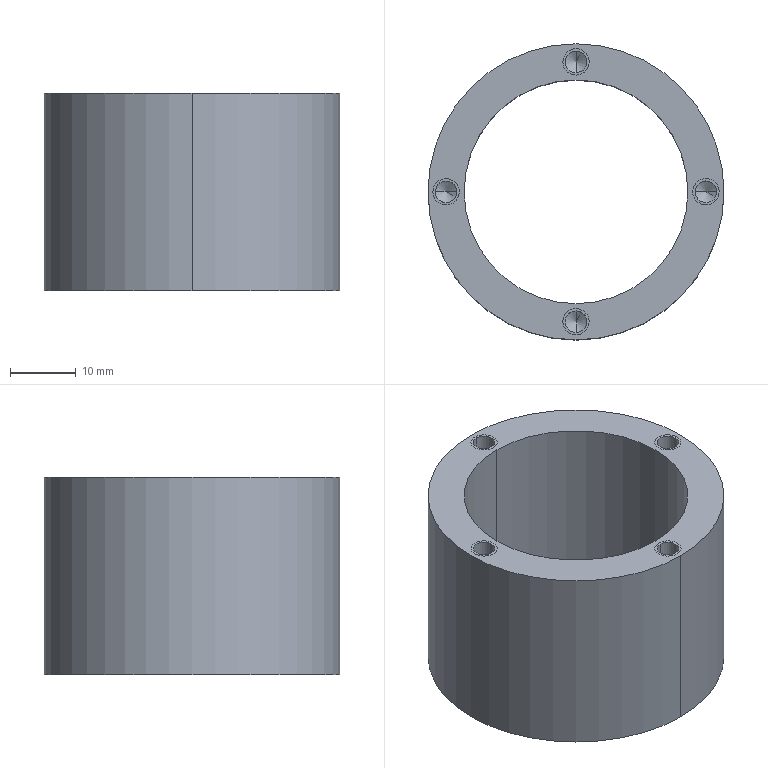CAM job | Mastercam | mm | 1 operations | part box 45 x 45 x 30
1. Drill/Counterbore | 7 - 4 倒角刀